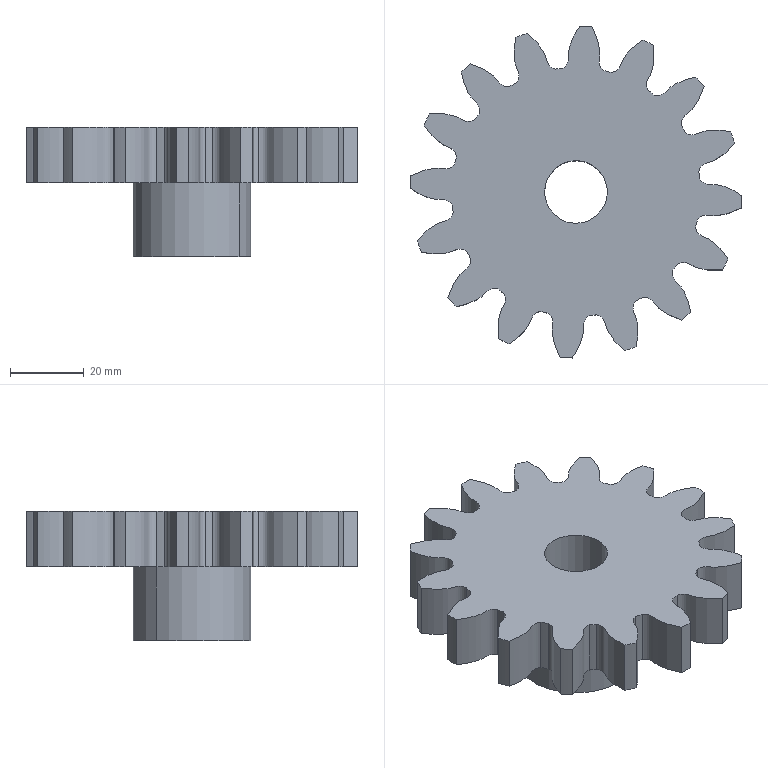Component | SolidWorks | Part21-2 | 1 solid | 71 faces | volume 81990 mm3 | cylinder 36 | spline 32 | plane 3 | commonest cylinder face diameters 90 x16 67.5 x16 17 x2 32 x2